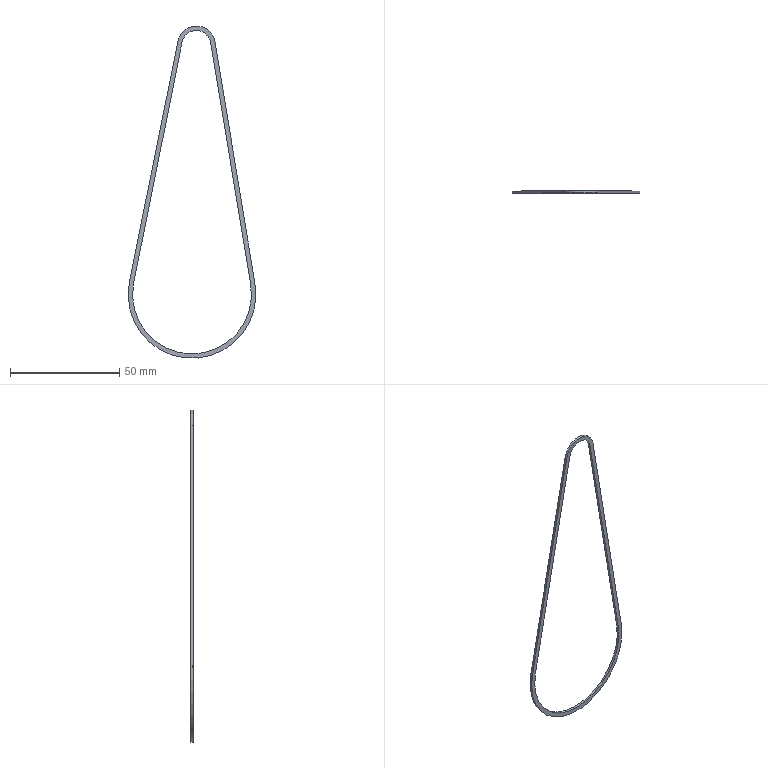Component | NX | MODEL9 | 1 solid | 13 faces | box 58.43 x 1 x 152.1 mm | volume 690 mm3 | plane 9 | cylinder 4 | commonest cylinder face diameters 13.245 x1 58.434 x1 17.245 x1 54.434 x1
STEP:
#1=CARTESIAN_POINT('',(0.,0.,0.));
#2=DIRECTION('',(0.,0.,1.));
#3=DIRECTION('',(1.,0.,0.));
#4=AXIS2_PLACEMENT_3D('',#1,#2,#3);
#5=CARTESIAN_POINT('',(-28.676,9.953,-108.889));
#6=VERTEX_POINT('',#5);
#7=CARTESIAN_POINT('',(-28.77,9.953,-109.381));
#8=VERTEX_POINT('',#7);
#9=CARTESIAN_POINT('',(-28.676,9.953,-108.889));
#10=DIRECTION('',(-0.1883,0.,-0.9821));
#11=VECTOR('',#10,1.);
#12=LINE('',#9,#11);
#13=CARTESIAN_POINT('',(-28.676,8.953,-108.889));
#14=DIRECTION('',(0.9821,0.,-0.1883));
#15=DIRECTION('',(0.1883,0.,0.9821));
#16=AXIS2_PLACEMENT_3D('',#13,#14,#15);
#17=PLANE('',#16);
#18=CARTESIAN_POINT('',(0.,-1.));
#19=DIRECTION('',(-1.,0.));
#20=VECTOR('',#19,1.);
#21=LINE('',#18,#20);
#22=(GEOMETRIC_REPRESENTATION_CONTEXT(2)PARAMETRIC_REPRESENTATION_CONTEXT()REPRESENTATION_CONTEXT('',''));
#23=DEFINITIONAL_REPRESENTATION('',(#21),#22);
#24=PCURVE('',#17,#23);
#25=CARTESIAN_POINT('',(-1.994,9.953,-114.26));
#26=DIRECTION('',(0.,-1.,0.));
#27=DIRECTION('',(1.,0.,0.));
#28=AXIS2_PLACEMENT_3D('',#25,#26,#27);
#29=PLANE('',#28);
#30=CARTESIAN_POINT('',(-26.682,5.371));
#31=DIRECTION('',(-0.1883,-0.9821));
#32=VECTOR('',#31,1.);
#33=LINE('',#30,#32);
#34=(GEOMETRIC_REPRESENTATION_CONTEXT(2)PARAMETRIC_REPRESENTATION_CONTEXT()REPRESENTATION_CONTEXT('',''));
#35=DEFINITIONAL_REPRESENTATION('',(#33),#34);
#36=PCURVE('',#29,#35);
#37=SURFACE_CURVE('',#12,(#24,#36),.PCURVE_S1.);
#38=EDGE_CURVE('',#6,#8,#37,.T.);
#39=ORIENTED_EDGE('',*,*,#38,.F.);
#40=CARTESIAN_POINT('',(-28.676,8.953,-108.889));
#41=VERTEX_POINT('',#40);
#42=CARTESIAN_POINT('',(-28.676,8.953,-108.889));
#43=DIRECTION('',(0.,1.,0.));
#44=VECTOR('',#43,1.);
#45=LINE('',#42,#44);
#46=CARTESIAN_POINT('',(0.,0.));
#47=DIRECTION('',(0.,-1.));
#48=VECTOR('',#47,1.);
#49=LINE('',#46,#48);
#50=(GEOMETRIC_REPRESENTATION_CONTEXT(2)PARAMETRIC_REPRESENTATION_CONTEXT()REPRESENTATION_CONTEXT('',''));
#51=DEFINITIONAL_REPRESENTATION('',(#49),#50);
#52=PCURVE('',#17,#51);
#53=CARTESIAN_POINT('',(-6.492,8.953,1.307));
#54=DIRECTION('',(0.9803,0.,-0.1974));
#55=DIRECTION('',(0.1974,0.,0.9803));
#56=AXIS2_PLACEMENT_3D('',#53,#54,#55);
#57=PLANE('',#56);
#58=CARTESIAN_POINT('',(-112.407,0.));
#59=DIRECTION('',(0.,-1.));
#60=VECTOR('',#59,1.);
#61=LINE('',#58,#60);
#62=(GEOMETRIC_REPRESENTATION_CONTEXT(2)PARAMETRIC_REPRESENTATION_CONTEXT()REPRESENTATION_CONTEXT('',''));
#63=DEFINITIONAL_REPRESENTATION('',(#61),#62);
#64=PCURVE('',#57,#63);
#65=SURFACE_CURVE('',#45,(#52,#64),.PCURVE_S1.);
#66=EDGE_CURVE('',#41,#6,#65,.T.);
#67=ORIENTED_EDGE('',*,*,#66,.F.);
#68=CARTESIAN_POINT('',(-28.77,8.953,-109.381));
#69=VERTEX_POINT('',#68);
#70=CARTESIAN_POINT('',(-28.676,8.953,-108.889));
#71=DIRECTION('',(-0.1883,0.,-0.9821));
#72=VECTOR('',#71,1.);
#73=LINE('',#70,#72);
#74=CARTESIAN_POINT('',(0.,0.));
#75=DIRECTION('',(-1.,0.));
#76=VECTOR('',#75,1.);
#77=LINE('',#74,#76);
#78=(GEOMETRIC_REPRESENTATION_CONTEXT(2)PARAMETRIC_REPRESENTATION_CONTEXT()REPRESENTATION_CONTEXT('',''));
#79=DEFINITIONAL_REPRESENTATION('',(#77),#78);
#80=PCURVE('',#17,#79);
#81=CARTESIAN_POINT('',(-1.994,8.953,-114.26));
#82=DIRECTION('',(0.,-1.,0.));
#83=DIRECTION('',(1.,0.,0.));
#84=AXIS2_PLACEMENT_3D('',#81,#82,#83);
#85=PLANE('',#84);
#86=CARTESIAN_POINT('',(-26.682,5.371));
#87=DIRECTION('',(-0.1883,-0.9821));
#88=VECTOR('',#87,1.);
#89=LINE('',#86,#88);
#90=(GEOMETRIC_REPRESENTATION_CONTEXT(2)PARAMETRIC_REPRESENTATION_CONTEXT()REPRESENTATION_CONTEXT('',''));
#91=DEFINITIONAL_REPRESENTATION('',(#89),#90);
#92=PCURVE('',#85,#91);
#93=SURFACE_CURVE('',#73,(#80,#92),.PCURVE_S1.);
#94=EDGE_CURVE('',#41,#69,#93,.T.);
#95=ORIENTED_EDGE('',*,*,#94,.T.);
#96=CARTESIAN_POINT('',(-28.77,8.953,-109.381));
#97=DIRECTION('',(0.,1.,0.));
#98=VECTOR('',#97,1.);
#99=LINE('',#96,#98);
#100=CARTESIAN_POINT('',(-0.5007,0.));
#101=DIRECTION('',(0.,-1.));
#102=VECTOR('',#101,1.);
#103=LINE('',#100,#102);
#104=(GEOMETRIC_REPRESENTATION_CONTEXT(2)PARAMETRIC_REPRESENTATION_CONTEXT()REPRESENTATION_CONTEXT('',''));
#105=DEFINITIONAL_REPRESENTATION('',(#103),#104);
#106=PCURVE('',#17,#105);
#107=CARTESIAN_POINT('',(-1.994,8.953,-114.26));
#108=DIRECTION('',(0.,1.,0.));
#109=DIRECTION('',(-1.,0.,0.));
#110=AXIS2_PLACEMENT_3D('',#107,#108,#109);
#111=CYLINDRICAL_SURFACE('',#110,27.217);
#112=CARTESIAN_POINT('',(6.463,0.));
#113=DIRECTION('',(0.,1.));
#114=VECTOR('',#113,1.);
#115=LINE('',#112,#114);
#116=(GEOMETRIC_REPRESENTATION_CONTEXT(2)PARAMETRIC_REPRESENTATION_CONTEXT()REPRESENTATION_CONTEXT('',''));
#117=DEFINITIONAL_REPRESENTATION('',(#115),#116);
#118=PCURVE('',#111,#117);
#119=SURFACE_CURVE('',#99,(#106,#118),.PCURVE_S1.);
#120=EDGE_CURVE('',#69,#8,#119,.T.);
#121=ORIENTED_EDGE('',*,*,#120,.T.);
#122=EDGE_LOOP('',(#39,#67,#95,#121));
#123=FACE_BOUND('',#122,.T.);
#124=ADVANCED_FACE('',(#123),#17,.T.);
#125=CARTESIAN_POINT('',(-6.492,9.953,1.307));
#126=VERTEX_POINT('',#125);
#127=CARTESIAN_POINT('',(-6.492,9.953,1.307));
#128=DIRECTION('',(-0.1974,0.,-0.9803));
#129=VECTOR('',#128,1.);
#130=LINE('',#127,#129);
#131=CARTESIAN_POINT('',(0.,-1.));
#132=DIRECTION('',(-1.,0.));
#133=VECTOR('',#132,1.);
#134=LINE('',#131,#133);
#135=(GEOMETRIC_REPRESENTATION_CONTEXT(2)PARAMETRIC_REPRESENTATION_CONTEXT()REPRESENTATION_CONTEXT('',''));
#136=DEFINITIONAL_REPRESENTATION('',(#134),#135);
#137=PCURVE('',#57,#136);
#138=CARTESIAN_POINT('',(-4.498,115.567));
#139=DIRECTION('',(-0.1974,-0.9803));
#140=VECTOR('',#139,1.);
#141=LINE('',#138,#140);
#142=(GEOMETRIC_REPRESENTATION_CONTEXT(2)PARAMETRIC_REPRESENTATION_CONTEXT()REPRESENTATION_CONTEXT('',''));
#143=DEFINITIONAL_REPRESENTATION('',(#141),#142);
#144=PCURVE('',#29,#143);
#145=SURFACE_CURVE('',#130,(#137,#144),.PCURVE_S1.);
#146=EDGE_CURVE('',#126,#6,#145,.T.);
#147=ORIENTED_EDGE('',*,*,#146,.F.);
#148=CARTESIAN_POINT('',(-6.492,8.953,1.307));
#149=VERTEX_POINT('',#148);
#150=CARTESIAN_POINT('',(-6.492,8.953,1.307));
#151=DIRECTION('',(0.,1.,0.));
#152=VECTOR('',#151,1.);
#153=LINE('',#150,#152);
#154=CARTESIAN_POINT('',(-0.,0.));
#155=DIRECTION('',(0.,-1.));
#156=VECTOR('',#155,1.);
#157=LINE('',#154,#156);
#158=(GEOMETRIC_REPRESENTATION_CONTEXT(2)PARAMETRIC_REPRESENTATION_CONTEXT()REPRESENTATION_CONTEXT('',''));
#159=DEFINITIONAL_REPRESENTATION('',(#157),#158);
#160=PCURVE('',#57,#159);
#161=CARTESIAN_POINT('',(0.,8.953,0.));
#162=DIRECTION('',(0.,1.,0.));
#163=DIRECTION('',(-1.,0.,0.));
#164=AXIS2_PLACEMENT_3D('',#161,#162,#163);
#165=CYLINDRICAL_SURFACE('',#164,6.622);
#166=CARTESIAN_POINT('',(0.1987,0.));
#167=DIRECTION('',(0.,1.));
#168=VECTOR('',#167,1.);
#169=LINE('',#166,#168);
#170=(GEOMETRIC_REPRESENTATION_CONTEXT(2)PARAMETRIC_REPRESENTATION_CONTEXT()REPRESENTATION_CONTEXT('',''));
#171=DEFINITIONAL_REPRESENTATION('',(#169),#170);
#172=PCURVE('',#165,#171);
#173=SURFACE_CURVE('',#153,(#160,#172),.PCURVE_S1.);
#174=EDGE_CURVE('',#149,#126,#173,.T.);
#175=ORIENTED_EDGE('',*,*,#174,.F.);
#176=CARTESIAN_POINT('',(-6.492,8.953,1.307));
#177=DIRECTION('',(-0.1974,0.,-0.9803));
#178=VECTOR('',#177,1.);
#179=LINE('',#176,#178);
#180=CARTESIAN_POINT('',(0.,0.));
#181=DIRECTION('',(-1.,0.));
#182=VECTOR('',#181,1.);
#183=LINE('',#180,#182);
#184=(GEOMETRIC_REPRESENTATION_CONTEXT(2)PARAMETRIC_REPRESENTATION_CONTEXT()REPRESENTATION_CONTEXT('',''));
#185=DEFINITIONAL_REPRESENTATION('',(#183),#184);
#186=PCURVE('',#57,#185);
#187=CARTESIAN_POINT('',(-4.498,115.567));
#188=DIRECTION('',(-0.1974,-0.9803));
#189=VECTOR('',#188,1.);
#190=LINE('',#187,#189);
#191=(GEOMETRIC_REPRESENTATION_CONTEXT(2)PARAMETRIC_REPRESENTATION_CONTEXT()REPRESENTATION_CONTEXT('',''));
#192=DEFINITIONAL_REPRESENTATION('',(#190),#191);
#193=PCURVE('',#85,#192);
#194=SURFACE_CURVE('',#179,(#186,#193),.PCURVE_S1.);
#195=EDGE_CURVE('',#149,#41,#194,.T.);
#196=ORIENTED_EDGE('',*,*,#195,.T.);
#197=ORIENTED_EDGE('',*,*,#66,.T.);
#198=EDGE_LOOP('',(#147,#175,#196,#197));
#199=FACE_BOUND('',#198,.T.);
#200=ADVANCED_FACE('',(#199),#57,.T.);
#201=ORIENTED_EDGE('',*,*,#174,.F.);
#202=CARTESIAN_POINT('',(6.534,8.953,1.08));
#203=VERTEX_POINT('',#202);
#204=CARTESIAN_POINT('',(0.,8.953,0.));
#205=DIRECTION('',(0.,-1.,0.));
#206=DIRECTION('',(1.,0.,0.));
#207=AXIS2_PLACEMENT_3D('',#204,#205,#206);
#208=CIRCLE('',#207,6.622);
#209=CARTESIAN_POINT('',(3.142,0.));
#210=DIRECTION('',(-1.,0.));
#211=VECTOR('',#210,1.);
#212=LINE('',#209,#211);
#213=(GEOMETRIC_REPRESENTATION_CONTEXT(2)PARAMETRIC_REPRESENTATION_CONTEXT()REPRESENTATION_CONTEXT('',''));
#214=DEFINITIONAL_REPRESENTATION('',(#212),#213);
#215=PCURVE('',#165,#214);
#216=CARTESIAN_POINT('',(1.994,114.26));
#217=DIRECTION('',(1.,0.));
#218=AXIS2_PLACEMENT_2D('',#216,#217);
#219=CIRCLE('',#218,6.622);
#220=(GEOMETRIC_REPRESENTATION_CONTEXT(2)PARAMETRIC_REPRESENTATION_CONTEXT()REPRESENTATION_CONTEXT('',''));
#221=DEFINITIONAL_REPRESENTATION('',(#219),#220);
#222=PCURVE('',#85,#221);
#223=SURFACE_CURVE('',#208,(#215,#222),.PCURVE_S1.);
#224=EDGE_CURVE('',#203,#149,#223,.T.);
#225=ORIENTED_EDGE('',*,*,#224,.F.);
#226=CARTESIAN_POINT('',(6.534,9.953,1.08));
#227=VERTEX_POINT('',#226);
#228=CARTESIAN_POINT('',(6.534,8.953,1.08));
#229=DIRECTION('',(0.,1.,0.));
#230=VECTOR('',#229,1.);
#231=LINE('',#228,#230);
#232=CARTESIAN_POINT('',(2.978,0.));
#233=DIRECTION('',(0.,1.));
#234=VECTOR('',#233,1.);
#235=LINE('',#232,#234);
#236=(GEOMETRIC_REPRESENTATION_CONTEXT(2)PARAMETRIC_REPRESENTATION_CONTEXT()REPRESENTATION_CONTEXT('',''));
#237=DEFINITIONAL_REPRESENTATION('',(#235),#236);
#238=PCURVE('',#165,#237);
#239=CARTESIAN_POINT('',(24.858,8.953,-109.823));
#240=DIRECTION('',(-0.9866,0.,-0.163));
#241=DIRECTION('',(0.163,0.,-0.9866));
#242=AXIS2_PLACEMENT_3D('',#239,#240,#241);
#243=PLANE('',#242);
#244=CARTESIAN_POINT('',(-112.407,0.));
#245=DIRECTION('',(0.,-1.));
#246=VECTOR('',#245,1.);
#247=LINE('',#244,#246);
#248=(GEOMETRIC_REPRESENTATION_CONTEXT(2)PARAMETRIC_REPRESENTATION_CONTEXT()REPRESENTATION_CONTEXT('',''));
#249=DEFINITIONAL_REPRESENTATION('',(#247),#248);
#250=PCURVE('',#243,#249);
#251=SURFACE_CURVE('',#231,(#238,#250),.PCURVE_S1.);
#252=EDGE_CURVE('',#203,#227,#251,.T.);
#253=ORIENTED_EDGE('',*,*,#252,.T.);
#254=CARTESIAN_POINT('',(0.,9.953,0.));
#255=DIRECTION('',(0.,-1.,0.));
#256=DIRECTION('',(1.,0.,0.));
#257=AXIS2_PLACEMENT_3D('',#254,#255,#256);
#258=CIRCLE('',#257,6.622);
#259=CARTESIAN_POINT('',(3.142,1.));
#260=DIRECTION('',(-1.,0.));
#261=VECTOR('',#260,1.);
#262=LINE('',#259,#261);
#263=(GEOMETRIC_REPRESENTATION_CONTEXT(2)PARAMETRIC_REPRESENTATION_CONTEXT()REPRESENTATION_CONTEXT('',''));
#264=DEFINITIONAL_REPRESENTATION('',(#262),#263);
#265=PCURVE('',#165,#264);
#266=CARTESIAN_POINT('',(1.994,114.26));
#267=DIRECTION('',(1.,0.));
#268=AXIS2_PLACEMENT_2D('',#266,#267);
#269=CIRCLE('',#268,6.622);
#270=(GEOMETRIC_REPRESENTATION_CONTEXT(2)PARAMETRIC_REPRESENTATION_CONTEXT()REPRESENTATION_CONTEXT('',''));
#271=DEFINITIONAL_REPRESENTATION('',(#269),#270);
#272=PCURVE('',#29,#271);
#273=SURFACE_CURVE('',#258,(#265,#272),.PCURVE_S1.);
#274=EDGE_CURVE('',#227,#126,#273,.T.);
#275=ORIENTED_EDGE('',*,*,#274,.T.);
#276=EDGE_LOOP('',(#201,#225,#253,#275));
#277=FACE_BOUND('',#276,.F.);
#278=ADVANCED_FACE('',(#277),#165,.F.);
#279=CARTESIAN_POINT('',(24.858,9.953,-109.823));
#280=VERTEX_POINT('',#279);
#281=CARTESIAN_POINT('',(24.858,9.953,-109.823));
#282=DIRECTION('',(-0.163,0.,0.9866));
#283=VECTOR('',#282,1.);
#284=LINE('',#281,#283);
#285=CARTESIAN_POINT('',(0.,-1.));
#286=DIRECTION('',(-1.,0.));
#287=VECTOR('',#286,1.);
#288=LINE('',#285,#287);
#289=(GEOMETRIC_REPRESENTATION_CONTEXT(2)PARAMETRIC_REPRESENTATION_CONTEXT()REPRESENTATION_CONTEXT('',''));
#290=DEFINITIONAL_REPRESENTATION('',(#288),#289);
#291=PCURVE('',#243,#290);
#292=CARTESIAN_POINT('',(26.853,4.437));
#293=DIRECTION('',(-0.163,0.9866));
#294=VECTOR('',#293,1.);
#295=LINE('',#292,#294);
#296=(GEOMETRIC_REPRESENTATION_CONTEXT(2)PARAMETRIC_REPRESENTATION_CONTEXT()REPRESENTATION_CONTEXT('',''));
#297=DEFINITIONAL_REPRESENTATION('',(#295),#296);
#298=PCURVE('',#29,#297);
#299=SURFACE_CURVE('',#284,(#291,#298),.PCURVE_S1.);
#300=EDGE_CURVE('',#280,#227,#299,.T.);
#301=ORIENTED_EDGE('',*,*,#300,.F.);
#302=CARTESIAN_POINT('',(24.858,8.953,-109.823));
#303=VERTEX_POINT('',#302);
#304=CARTESIAN_POINT('',(24.858,8.953,-109.823));
#305=DIRECTION('',(0.,1.,0.));
#306=VECTOR('',#305,1.);
#307=LINE('',#304,#306);
#308=CARTESIAN_POINT('',(0.,0.));
#309=DIRECTION('',(0.,-1.));
#310=VECTOR('',#309,1.);
#311=LINE('',#308,#310);
#312=(GEOMETRIC_REPRESENTATION_CONTEXT(2)PARAMETRIC_REPRESENTATION_CONTEXT()REPRESENTATION_CONTEXT('',''));
#313=DEFINITIONAL_REPRESENTATION('',(#311),#312);
#314=PCURVE('',#243,#313);
#315=CARTESIAN_POINT('',(2.978,0.));
#316=DIRECTION('',(0.,1.));
#317=VECTOR('',#316,1.);
#318=LINE('',#315,#317);
#319=(GEOMETRIC_REPRESENTATION_CONTEXT(2)PARAMETRIC_REPRESENTATION_CONTEXT()REPRESENTATION_CONTEXT('',''));
#320=DEFINITIONAL_REPRESENTATION('',(#318),#319);
#321=PCURVE('',#111,#320);
#322=SURFACE_CURVE('',#307,(#314,#321),.PCURVE_S1.);
#323=EDGE_CURVE('',#303,#280,#322,.T.);
#324=ORIENTED_EDGE('',*,*,#323,.F.);
#325=CARTESIAN_POINT('',(24.858,8.953,-109.823));
#326=DIRECTION('',(-0.163,0.,0.9866));
#327=VECTOR('',#326,1.);
#328=LINE('',#325,#327);
#329=CARTESIAN_POINT('',(0.,0.));
#330=DIRECTION('',(-1.,0.));
#331=VECTOR('',#330,1.);
#332=LINE('',#329,#331);
#333=(GEOMETRIC_REPRESENTATION_CONTEXT(2)PARAMETRIC_REPRESENTATION_CONTEXT()REPRESENTATION_CONTEXT('',''));
#334=DEFINITIONAL_REPRESENTATION('',(#332),#333);
#335=PCURVE('',#243,#334);
#336=CARTESIAN_POINT('',(26.853,4.437));
#337=DIRECTION('',(-0.163,0.9866));
#338=VECTOR('',#337,1.);
#339=LINE('',#336,#338);
#340=(GEOMETRIC_REPRESENTATION_CONTEXT(2)PARAMETRIC_REPRESENTATION_CONTEXT()REPRESENTATION_CONTEXT('',''));
#341=DEFINITIONAL_REPRESENTATION('',(#339),#340);
#342=PCURVE('',#85,#341);
#343=SURFACE_CURVE('',#328,(#335,#342),.PCURVE_S1.);
#344=EDGE_CURVE('',#303,#203,#343,.T.);
#345=ORIENTED_EDGE('',*,*,#344,.T.);
#346=ORIENTED_EDGE('',*,*,#252,.T.);
#347=EDGE_LOOP('',(#301,#324,#345,#346));
#348=FACE_BOUND('',#347,.T.);
#349=ADVANCED_FACE('',(#348),#243,.T.);
#350=CARTESIAN_POINT('',(-8.453,9.953,1.702));
#351=VERTEX_POINT('',#350);
#352=CARTESIAN_POINT('',(-30.639,9.953,-108.503));
#353=VERTEX_POINT('',#352);
#354=CARTESIAN_POINT('',(-8.453,9.953,1.702));
#355=DIRECTION('',(-0.1974,0.,-0.9803));
#356=VECTOR('',#355,1.);
#357=LINE('',#354,#356);
#358=CARTESIAN_POINT('',(-8.453,8.953,1.702));
#359=DIRECTION('',(0.9803,0.,-0.1974));
#360=DIRECTION('',(0.1974,0.,0.9803));
#361=AXIS2_PLACEMENT_3D('',#358,#359,#360);
#362=PLANE('',#361);
#363=CARTESIAN_POINT('',(0.,-1.));
#364=DIRECTION('',(-1.,0.));
#365=VECTOR('',#364,1.);
#366=LINE('',#363,#365);
#367=(GEOMETRIC_REPRESENTATION_CONTEXT(2)PARAMETRIC_REPRESENTATION_CONTEXT()REPRESENTATION_CONTEXT('',''));
#368=DEFINITIONAL_REPRESENTATION('',(#366),#367);
#369=PCURVE('',#362,#368);
#370=CARTESIAN_POINT('',(-6.458,115.962));
#371=DIRECTION('',(-0.1974,-0.9803));
#372=VECTOR('',#371,1.);
#373=LINE('',#370,#372);
#374=(GEOMETRIC_REPRESENTATION_CONTEXT(2)PARAMETRIC_REPRESENTATION_CONTEXT()REPRESENTATION_CONTEXT('',''));
#375=DEFINITIONAL_REPRESENTATION('',(#373),#374);
#376=PCURVE('',#29,#375);
#377=SURFACE_CURVE('',#357,(#369,#376),.PCURVE_S1.);
#378=EDGE_CURVE('',#351,#353,#377,.T.);
#379=ORIENTED_EDGE('',*,*,#378,.T.);
#380=CARTESIAN_POINT('',(-30.639,8.953,-108.503));
#381=VERTEX_POINT('',#380);
#382=CARTESIAN_POINT('',(-30.639,8.953,-108.503));
#383=DIRECTION('',(0.,1.,0.));
#384=VECTOR('',#383,1.);
#385=LINE('',#382,#384);
#386=CARTESIAN_POINT('',(-112.416,0.));
#387=DIRECTION('',(0.,-1.));
#388=VECTOR('',#387,1.);
#389=LINE('',#386,#388);
#390=(GEOMETRIC_REPRESENTATION_CONTEXT(2)PARAMETRIC_REPRESENTATION_CONTEXT()REPRESENTATION_CONTEXT('',''));
#391=DEFINITIONAL_REPRESENTATION('',(#389),#390);
#392=PCURVE('',#362,#391);
#393=CARTESIAN_POINT('',(-30.639,8.953,-108.503));
#394=DIRECTION('',(0.9821,0.,-0.1883));
#395=DIRECTION('',(0.1883,0.,0.9821));
#396=AXIS2_PLACEMENT_3D('',#393,#394,#395);
#397=PLANE('',#396);
#398=CARTESIAN_POINT('',(0.,0.));
#399=DIRECTION('',(0.,-1.));
#400=VECTOR('',#399,1.);
#401=LINE('',#398,#400);
#402=(GEOMETRIC_REPRESENTATION_CONTEXT(2)PARAMETRIC_REPRESENTATION_CONTEXT()REPRESENTATION_CONTEXT('',''));
#403=DEFINITIONAL_REPRESENTATION('',(#401),#402);
#404=PCURVE('',#397,#403);
#405=SURFACE_CURVE('',#385,(#392,#404),.PCURVE_S1.);
#406=EDGE_CURVE('',#381,#353,#405,.T.);
#407=ORIENTED_EDGE('',*,*,#406,.F.);
#408=CARTESIAN_POINT('',(-8.453,8.953,1.702));
#409=VERTEX_POINT('',#408);
#410=CARTESIAN_POINT('',(-8.453,8.953,1.702));
#411=DIRECTION('',(-0.1974,0.,-0.9803));
#412=VECTOR('',#411,1.);
#413=LINE('',#410,#412);
#414=CARTESIAN_POINT('',(0.,0.));
#415=DIRECTION('',(-1.,0.));
#416=VECTOR('',#415,1.);
#417=LINE('',#414,#416);
#418=(GEOMETRIC_REPRESENTATION_CONTEXT(2)PARAMETRIC_REPRESENTATION_CONTEXT()REPRESENTATION_CONTEXT('',''));
#419=DEFINITIONAL_REPRESENTATION('',(#417),#418);
#420=PCURVE('',#362,#419);
#421=CARTESIAN_POINT('',(-6.458,115.962));
#422=DIRECTION('',(-0.1974,-0.9803));
#423=VECTOR('',#422,1.);
#424=LINE('',#421,#423);
#425=(GEOMETRIC_REPRESENTATION_CONTEXT(2)PARAMETRIC_REPRESENTATION_CONTEXT()REPRESENTATION_CONTEXT('',''));
#426=DEFINITIONAL_REPRESENTATION('',(#424),#425);
#427=PCURVE('',#85,#426);
#428=SURFACE_CURVE('',#413,(#420,#427),.PCURVE_S1.);
#429=EDGE_CURVE('',#409,#381,#428,.T.);
#430=ORIENTED_EDGE('',*,*,#429,.F.);
#431=CARTESIAN_POINT('',(-8.453,8.953,1.702));
#432=DIRECTION('',(0.,1.,0.));
#433=VECTOR('',#432,1.);
#434=LINE('',#431,#433);
#435=CARTESIAN_POINT('',(0.,0.));
#436=DIRECTION('',(0.,-1.));
#437=VECTOR('',#436,1.);
#438=LINE('',#435,#437);
#439=(GEOMETRIC_REPRESENTATION_CONTEXT(2)PARAMETRIC_REPRESENTATION_CONTEXT()REPRESENTATION_CONTEXT('',''));
#440=DEFINITIONAL_REPRESENTATION('',(#438),#439);
#441=PCURVE('',#362,#440);
#442=CARTESIAN_POINT('',(0.,8.953,0.));
#443=DIRECTION('',(0.,1.,0.));
#444=DIRECTION('',(-1.,0.,0.));
#445=AXIS2_PLACEMENT_3D('',#442,#443,#444);
#446=CYLINDRICAL_SURFACE('',#445,8.623);
#447=CARTESIAN_POINT('',(0.1987,0.));
#448=DIRECTION('',(0.,1.));
#449=VECTOR('',#448,1.);
#450=LINE('',#447,#449);
#451=(GEOMETRIC_REPRESENTATION_CONTEXT(2)PARAMETRIC_REPRESENTATION_CONTEXT()REPRESENTATION_CONTEXT('',''));
#452=DEFINITIONAL_REPRESENTATION('',(#450),#451);
#453=PCURVE('',#446,#452);
#454=SURFACE_CURVE('',#434,(#441,#453),.PCURVE_S1.);
#455=EDGE_CURVE('',#409,#351,#454,.T.);
#456=ORIENTED_EDGE('',*,*,#455,.T.);
#457=EDGE_LOOP('',(#379,#407,#430,#456));
#458=FACE_BOUND('',#457,.T.);
#459=ADVANCED_FACE('',(#458),#362,.F.);
#460=CARTESIAN_POINT('',(-30.736,9.953,-109.013));
#461=VERTEX_POINT('',#460);
#462=CARTESIAN_POINT('',(-30.639,9.953,-108.503));
#463=DIRECTION('',(-0.1883,0.,-0.9821));
#464=VECTOR('',#463,1.);
#465=LINE('',#462,#464);
#466=CARTESIAN_POINT('',(0.,-1.));
#467=DIRECTION('',(-1.,0.));
#468=VECTOR('',#467,1.);
#469=LINE('',#466,#468);
#470=(GEOMETRIC_REPRESENTATION_CONTEXT(2)PARAMETRIC_REPRESENTATION_CONTEXT()REPRESENTATION_CONTEXT('',''));
#471=DEFINITIONAL_REPRESENTATION('',(#469),#470);
#472=PCURVE('',#397,#471);
#473=CARTESIAN_POINT('',(-28.644,5.757));
#474=DIRECTION('',(-0.1883,-0.9821));
#475=VECTOR('',#474,1.);
#476=LINE('',#473,#475);
#477=(GEOMETRIC_REPRESENTATION_CONTEXT(2)PARAMETRIC_REPRESENTATION_CONTEXT()REPRESENTATION_CONTEXT('',''));
#478=DEFINITIONAL_REPRESENTATION('',(#476),#477);
#479=PCURVE('',#29,#478);
#480=SURFACE_CURVE('',#465,(#472,#479),.PCURVE_S1.);
#481=EDGE_CURVE('',#353,#461,#480,.T.);
#482=ORIENTED_EDGE('',*,*,#481,.T.);
#483=CARTESIAN_POINT('',(-30.736,8.953,-109.013));
#484=VERTEX_POINT('',#483);
#485=CARTESIAN_POINT('',(-30.736,8.953,-109.013));
#486=DIRECTION('',(0.,1.,0.));
#487=VECTOR('',#486,1.);
#488=LINE('',#485,#487);
#489=CARTESIAN_POINT('',(-0.5191,0.));
#490=DIRECTION('',(0.,-1.));
#491=VECTOR('',#490,1.);
#492=LINE('',#489,#491);
#493=(GEOMETRIC_REPRESENTATION_CONTEXT(2)PARAMETRIC_REPRESENTATION_CONTEXT()REPRESENTATION_CONTEXT('',''));
#494=DEFINITIONAL_REPRESENTATION('',(#492),#493);
#495=PCURVE('',#397,#494);
#496=CARTESIAN_POINT('',(-30.736,8.953,-109.013));
#497=DIRECTION('',(0.9838,0.,-0.1793));
#498=DIRECTION('',(0.1793,0.,0.9838));
#499=AXIS2_PLACEMENT_3D('',#496,#497,#498);
#500=PLANE('',#499);
#501=CARTESIAN_POINT('',(0.,0.));
#502=DIRECTION('',(0.,-1.));
#503=VECTOR('',#502,1.);
#504=LINE('',#501,#503);
#505=(GEOMETRIC_REPRESENTATION_CONTEXT(2)PARAMETRIC_REPRESENTATION_CONTEXT()REPRESENTATION_CONTEXT('',''));
#506=DEFINITIONAL_REPRESENTATION('',(#504),#505);
#507=PCURVE('',#500,#506);
#508=SURFACE_CURVE('',#488,(#495,#507),.PCURVE_S1.);
#509=EDGE_CURVE('',#484,#461,#508,.T.);
#510=ORIENTED_EDGE('',*,*,#509,.F.);
#511=CARTESIAN_POINT('',(-30.639,8.953,-108.503));
#512=DIRECTION('',(-0.1883,0.,-0.9821));
#513=VECTOR('',#512,1.);
#514=LINE('',#511,#513);
#515=CARTESIAN_POINT('',(0.,0.));
#516=DIRECTION('',(-1.,0.));
#517=VECTOR('',#516,1.);
#518=LINE('',#515,#517);
#519=(GEOMETRIC_REPRESENTATION_CONTEXT(2)PARAMETRIC_REPRESENTATION_CONTEXT()REPRESENTATION_CONTEXT('',''));
#520=DEFINITIONAL_REPRESENTATION('',(#518),#519);
#521=PCURVE('',#397,#520);
#522=CARTESIAN_POINT('',(-28.644,5.757));
#523=DIRECTION('',(-0.1883,-0.9821));
#524=VECTOR('',#523,1.);
#525=LINE('',#522,#524);
#526=(GEOMETRIC_REPRESENTATION_CONTEXT(2)PARAMETRIC_REPRESENTATION_CONTEXT()REPRESENTATION_CONTEXT('',''));
#527=DEFINITIONAL_REPRESENTATION('',(#525),#526);
#528=PCURVE('',#85,#527);
#529=SURFACE_CURVE('',#514,(#521,#528),.PCURVE_S1.);
#530=EDGE_CURVE('',#381,#484,#529,.T.);
#531=ORIENTED_EDGE('',*,*,#530,.F.);
#532=ORIENTED_EDGE('',*,*,#406,.T.);
#533=EDGE_LOOP('',(#482,#510,#531,#532));
#534=FACE_BOUND('',#533,.T.);
#535=ADVANCED_FACE('',(#534),#397,.F.);
#536=CARTESIAN_POINT('',(-30.738,9.953,-109.022));
#537=VERTEX_POINT('',#536);
#538=CARTESIAN_POINT('',(-30.736,9.953,-109.013));
#539=DIRECTION('',(-0.1793,0.,-0.9838));
#540=VECTOR('',#539,1.);
#541=LINE('',#538,#540);
#542=CARTESIAN_POINT('',(0.,-1.));
#543=DIRECTION('',(-1.,0.));
#544=VECTOR('',#543,1.);
#545=LINE('',#542,#544);
#546=(GEOMETRIC_REPRESENTATION_CONTEXT(2)PARAMETRIC_REPRESENTATION_CONTEXT()REPRESENTATION_CONTEXT('',''));
#547=DEFINITIONAL_REPRESENTATION('',(#545),#546);
#548=PCURVE('',#500,#547);
#549=CARTESIAN_POINT('',(-28.742,5.247));
#550=DIRECTION('',(-0.1793,-0.9838));
#551=VECTOR('',#550,1.);
#552=LINE('',#549,#551);
#553=(GEOMETRIC_REPRESENTATION_CONTEXT(2)PARAMETRIC_REPRESENTATION_CONTEXT()REPRESENTATION_CONTEXT('',''));
#554=DEFINITIONAL_REPRESENTATION('',(#552),#553);
#555=PCURVE('',#29,#554);
#556=SURFACE_CURVE('',#541,(#548,#555),.PCURVE_S1.);
#557=EDGE_CURVE('',#461,#537,#556,.T.);
#558=ORIENTED_EDGE('',*,*,#557,.T.);
#559=CARTESIAN_POINT('',(-30.738,8.953,-109.022));
#560=VERTEX_POINT('',#559);
#561=CARTESIAN_POINT('',(-30.738,8.953,-109.022));
#562=DIRECTION('',(0.,1.,0.));
#563=VECTOR('',#562,1.);
#564=LINE('',#561,#563);
#565=CARTESIAN_POINT('',(-0.009199,0.));
#566=DIRECTION('',(0.,-1.));
#567=VECTOR('',#566,1.);
#568=LINE('',#565,#567);
#569=(GEOMETRIC_REPRESENTATION_CONTEXT(2)PARAMETRIC_REPRESENTATION_CONTEXT()REPRESENTATION_CONTEXT('',''));
#570=DEFINITIONAL_REPRESENTATION('',(#568),#569);
#571=PCURVE('',#500,#570);
#572=CARTESIAN_POINT('',(-1.994,8.953,-114.26));
#573=DIRECTION('',(0.,1.,0.));
#574=DIRECTION('',(-1.,0.,0.));
#575=AXIS2_PLACEMENT_3D('',#572,#573,#574);
#576=CYLINDRICAL_SURFACE('',#575,29.217);
#577=CARTESIAN_POINT('',(6.463,0.));
#578=DIRECTION('',(0.,1.));
#579=VECTOR('',#578,1.);
#580=LINE('',#577,#579);
#581=(GEOMETRIC_REPRESENTATION_CONTEXT(2)PARAMETRIC_REPRESENTATION_CONTEXT()REPRESENTATION_CONTEXT('',''));
#582=DEFINITIONAL_REPRESENTATION('',(#580),#581);
#583=PCURVE('',#576,#582);
#584=SURFACE_CURVE('',#564,(#571,#583),.PCURVE_S1.);
#585=EDGE_CURVE('',#560,#537,#584,.T.);
#586=ORIENTED_EDGE('',*,*,#585,.F.);
#587=CARTESIAN_POINT('',(-30.736,8.953,-109.013));
#588=DIRECTION('',(-0.1793,0.,-0.9838));
#589=VECTOR('',#588,1.);
#590=LINE('',#587,#589);
#591=CARTESIAN_POINT('',(0.,0.));
#592=DIRECTION('',(-1.,0.));
#593=VECTOR('',#592,1.);
#594=LINE('',#591,#593);
#595=(GEOMETRIC_REPRESENTATION_CONTEXT(2)PARAMETRIC_REPRESENTATION_CONTEXT()REPRESENTATION_CONTEXT('',''));
#596=DEFINITIONAL_REPRESENTATION('',(#594),#595);
#597=PCURVE('',#500,#596);
#598=CARTESIAN_POINT('',(-28.742,5.247));
#599=DIRECTION('',(-0.1793,-0.9838));
#600=VECTOR('',#599,1.);
#601=LINE('',#598,#600);
#602=(GEOMETRIC_REPRESENTATION_CONTEXT(2)PARAMETRIC_REPRESENTATION_CONTEXT()REPRESENTATION_CONTEXT('',''));
#603=DEFINITIONAL_REPRESENTATION('',(#601),#602);
#604=PCURVE('',#85,#603);
#605=SURFACE_CURVE('',#590,(#597,#604),.PCURVE_S1.);
#606=EDGE_CURVE('',#484,#560,#605,.T.);
#607=ORIENTED_EDGE('',*,*,#606,.F.);
#608=ORIENTED_EDGE('',*,*,#509,.T.);
#609=EDGE_LOOP('',(#558,#586,#607,#608));
#610=FACE_BOUND('',#609,.T.);
#611=ADVANCED_FACE('',(#610),#500,.F.);
#612=CARTESIAN_POINT('',(26.832,9.953,-109.497));
#613=VERTEX_POINT('',#612);
#614=CARTESIAN_POINT('',(-1.994,9.953,-114.26));
#615=DIRECTION('',(0.,-1.,0.));
#616=DIRECTION('',(1.,0.,0.));
#617=AXIS2_PLACEMENT_3D('',#614,#615,#616);
#618=CIRCLE('',#617,29.217);
#619=CARTESIAN_POINT('',(9.425,1.));
#620=DIRECTION('',(-1.,0.));
#621=VECTOR('',#620,1.);
#622=LINE('',#619,#621);
#623=(GEOMETRIC_REPRESENTATION_CONTEXT(2)PARAMETRIC_REPRESENTATION_CONTEXT()REPRESENTATION_CONTEXT('',''));
#624=DEFINITIONAL_REPRESENTATION('',(#622),#623);
#625=PCURVE('',#576,#624);
#626=CARTESIAN_POINT('',(0.,0.));
#627=DIRECTION('',(1.,0.));
#628=AXIS2_PLACEMENT_2D('',#626,#627);
#629=CIRCLE('',#628,29.217);
#630=(GEOMETRIC_REPRESENTATION_CONTEXT(2)PARAMETRIC_REPRESENTATION_CONTEXT()REPRESENTATION_CONTEXT('',''));
#631=DEFINITIONAL_REPRESENTATION('',(#629),#630);
#632=PCURVE('',#29,#631);
#633=SURFACE_CURVE('',#618,(#625,#632),.PCURVE_S1.);
#634=EDGE_CURVE('',#537,#613,#633,.T.);
#635=ORIENTED_EDGE('',*,*,#634,.T.);
#636=CARTESIAN_POINT('',(26.832,8.953,-109.497));
#637=VERTEX_POINT('',#636);
#638=CARTESIAN_POINT('',(26.832,8.953,-109.497));
#639=DIRECTION('',(0.,1.,0.));
#640=VECTOR('',#639,1.);
#641=LINE('',#638,#640);
#642=CARTESIAN_POINT('',(2.978,0.));
#643=DIRECTION('',(0.,1.));
#644=VECTOR('',#643,1.);
#645=LINE('',#642,#644);
#646=(GEOMETRIC_REPRESENTATION_CONTEXT(2)PARAMETRIC_REPRESENTATION_CONTEXT()REPRESENTATION_CONTEXT('',''));
#647=DEFINITIONAL_REPRESENTATION('',(#645),#646);
#648=PCURVE('',#576,#647);
#649=CARTESIAN_POINT('',(26.832,8.953,-109.497));
#650=DIRECTION('',(-0.9866,0.,-0.163));
#651=DIRECTION('',(0.163,0.,-0.9866));
#652=AXIS2_PLACEMENT_3D('',#649,#650,#651);
#653=PLANE('',#652);
#654=CARTESIAN_POINT('',(0.,0.));
#655=DIRECTION('',(0.,-1.));
#656=VECTOR('',#655,1.);
#657=LINE('',#654,#656);
#658=(GEOMETRIC_REPRESENTATION_CONTEXT(2)PARAMETRIC_REPRESENTATION_CONTEXT()REPRESENTATION_CONTEXT('',''));
#659=DEFINITIONAL_REPRESENTATION('',(#657),#658);
#660=PCURVE('',#653,#659);
#661=SURFACE_CURVE('',#641,(#648,#660),.PCURVE_S1.);
#662=EDGE_CURVE('',#637,#613,#661,.T.);
#663=ORIENTED_EDGE('',*,*,#662,.F.);
#664=CARTESIAN_POINT('',(-1.994,8.953,-114.26));
#665=DIRECTION('',(0.,-1.,0.));
#666=DIRECTION('',(1.,0.,0.));
#667=AXIS2_PLACEMENT_3D('',#664,#665,#666);
#668=CIRCLE('',#667,29.217);
#669=CARTESIAN_POINT('',(9.425,0.));
#670=DIRECTION('',(-1.,0.));
#671=VECTOR('',#670,1.);
#672=LINE('',#669,#671);
#673=(GEOMETRIC_REPRESENTATION_CONTEXT(2)PARAMETRIC_REPRESENTATION_CONTEXT()REPRESENTATION_CONTEXT('',''));
#674=DEFINITIONAL_REPRESENTATION('',(#672),#673);
#675=PCURVE('',#576,#674);
#676=CARTESIAN_POINT('',(0.,0.));
#677=DIRECTION('',(1.,0.));
#678=AXIS2_PLACEMENT_2D('',#676,#677);
#679=CIRCLE('',#678,29.217);
#680=(GEOMETRIC_REPRESENTATION_CONTEXT(2)PARAMETRIC_REPRESENTATION_CONTEXT()REPRESENTATION_CONTEXT('',''));
#681=DEFINITIONAL_REPRESENTATION('',(#679),#680);
#682=PCURVE('',#85,#681);
#683=SURFACE_CURVE('',#668,(#675,#682),.PCURVE_S1.);
#684=EDGE_CURVE('',#560,#637,#683,.T.);
#685=ORIENTED_EDGE('',*,*,#684,.F.);
#686=ORIENTED_EDGE('',*,*,#585,.T.);
#687=EDGE_LOOP('',(#635,#663,#685,#686));
#688=FACE_BOUND('',#687,.T.);
#689=ADVANCED_FACE('',(#688),#576,.T.);
#690=CARTESIAN_POINT('',(8.507,9.953,1.406));
#691=VERTEX_POINT('',#690);
#692=CARTESIAN_POINT('',(26.832,9.953,-109.497));
#693=DIRECTION('',(-0.163,0.,0.9866));
#694=VECTOR('',#693,1.);
#695=LINE('',#692,#694);
#696=CARTESIAN_POINT('',(0.,-1.));
#697=DIRECTION('',(-1.,0.));
#698=VECTOR('',#697,1.);
#699=LINE('',#696,#698);
#700=(GEOMETRIC_REPRESENTATION_CONTEXT(2)PARAMETRIC_REPRESENTATION_CONTEXT()REPRESENTATION_CONTEXT('',''));
#701=DEFINITIONAL_REPRESENTATION('',(#699),#700);
#702=PCURVE('',#653,#701);
#703=CARTESIAN_POINT('',(28.826,4.763));
#704=DIRECTION('',(-0.163,0.9866));
#705=VECTOR('',#704,1.);
#706=LINE('',#703,#705);
#707=(GEOMETRIC_REPRESENTATION_CONTEXT(2)PARAMETRIC_REPRESENTATION_CONTEXT()REPRESENTATION_CONTEXT('',''));
#708=DEFINITIONAL_REPRESENTATION('',(#706),#707);
#709=PCURVE('',#29,#708);
#710=SURFACE_CURVE('',#695,(#702,#709),.PCURVE_S1.);
#711=EDGE_CURVE('',#613,#691,#710,.T.);
#712=ORIENTED_EDGE('',*,*,#711,.T.);
#713=CARTESIAN_POINT('',(8.507,8.953,1.406));
#714=VERTEX_POINT('',#713);
#715=CARTESIAN_POINT('',(8.507,8.953,1.406));
#716=DIRECTION('',(0.,1.,0.));
#717=VECTOR('',#716,1.);
#718=LINE('',#715,#717);
#719=CARTESIAN_POINT('',(-112.407,0.));
#720=DIRECTION('',(0.,-1.));
#721=VECTOR('',#720,1.);
#722=LINE('',#719,#721);
#723=(GEOMETRIC_REPRESENTATION_CONTEXT(2)PARAMETRIC_REPRESENTATION_CONTEXT()REPRESENTATION_CONTEXT('',''));
#724=DEFINITIONAL_REPRESENTATION('',(#722),#723);
#725=PCURVE('',#653,#724);
#726=CARTESIAN_POINT('',(2.978,0.));
#727=DIRECTION('',(0.,1.));
#728=VECTOR('',#727,1.);
#729=LINE('',#726,#728);
#730=(GEOMETRIC_REPRESENTATION_CONTEXT(2)PARAMETRIC_REPRESENTATION_CONTEXT()REPRESENTATION_CONTEXT('',''));
#731=DEFINITIONAL_REPRESENTATION('',(#729),#730);
#732=PCURVE('',#446,#731);
#733=SURFACE_CURVE('',#718,(#725,#732),.PCURVE_S1.);
#734=EDGE_CURVE('',#714,#691,#733,.T.);
#735=ORIENTED_EDGE('',*,*,#734,.F.);
#736=CARTESIAN_POINT('',(26.832,8.953,-109.497));
#737=DIRECTION('',(-0.163,0.,0.9866));
#738=VECTOR('',#737,1.);
#739=LINE('',#736,#738);
#740=CARTESIAN_POINT('',(0.,0.));
#741=DIRECTION('',(-1.,0.));
#742=VECTOR('',#741,1.);
#743=LINE('',#740,#742);
#744=(GEOMETRIC_REPRESENTATION_CONTEXT(2)PARAMETRIC_REPRESENTATION_CONTEXT()REPRESENTATION_CONTEXT('',''));
#745=DEFINITIONAL_REPRESENTATION('',(#743),#744);
#746=PCURVE('',#653,#745);
#747=CARTESIAN_POINT('',(28.826,4.763));
#748=DIRECTION('',(-0.163,0.9866));
#749=VECTOR('',#748,1.);
#750=LINE('',#747,#749);
#751=(GEOMETRIC_REPRESENTATION_CONTEXT(2)PARAMETRIC_REPRESENTATION_CONTEXT()REPRESENTATION_CONTEXT('',''));
#752=DEFINITIONAL_REPRESENTATION('',(#750),#751);
#753=PCURVE('',#85,#752);
#754=SURFACE_CURVE('',#739,(#746,#753),.PCURVE_S1.);
#755=EDGE_CURVE('',#637,#714,#754,.T.);
#756=ORIENTED_EDGE('',*,*,#755,.F.);
#757=ORIENTED_EDGE('',*,*,#662,.T.);
#758=EDGE_LOOP('',(#712,#735,#756,#757));
#759=FACE_BOUND('',#758,.T.);
#760=ADVANCED_FACE('',(#759),#653,.F.);
#761=CARTESIAN_POINT('',(0.,9.953,0.));
#762=DIRECTION('',(0.,-1.,0.));
#763=DIRECTION('',(1.,0.,0.));
#764=AXIS2_PLACEMENT_3D('',#761,#762,#763);
#765=CIRCLE('',#764,8.623);
#766=CARTESIAN_POINT('',(3.142,1.));
#767=DIRECTION('',(-1.,0.));
#768=VECTOR('',#767,1.);
#769=LINE('',#766,#768);
#770=(GEOMETRIC_REPRESENTATION_CONTEXT(2)PARAMETRIC_REPRESENTATION_CONTEXT()REPRESENTATION_CONTEXT('',''));
#771=DEFINITIONAL_REPRESENTATION('',(#769),#770);
#772=PCURVE('',#446,#771);
#773=CARTESIAN_POINT('',(1.994,114.26));
#774=DIRECTION('',(1.,0.));
#775=AXIS2_PLACEMENT_2D('',#773,#774);
#776=CIRCLE('',#775,8.623);
#777=(GEOMETRIC_REPRESENTATION_CONTEXT(2)PARAMETRIC_REPRESENTATION_CONTEXT()REPRESENTATION_CONTEXT('',''));
#778=DEFINITIONAL_REPRESENTATION('',(#776),#777);
#779=PCURVE('',#29,#778);
#780=SURFACE_CURVE('',#765,(#772,#779),.PCURVE_S1.);
#781=EDGE_CURVE('',#691,#351,#780,.T.);
#782=ORIENTED_EDGE('',*,*,#781,.T.);
#783=ORIENTED_EDGE('',*,*,#455,.F.);
#784=CARTESIAN_POINT('',(0.,8.953,0.));
#785=DIRECTION('',(0.,-1.,0.));
#786=DIRECTION('',(1.,0.,0.));
#787=AXIS2_PLACEMENT_3D('',#784,#785,#786);
#788=CIRCLE('',#787,8.623);
#789=CARTESIAN_POINT('',(3.142,0.));
#790=DIRECTION('',(-1.,0.));
#791=VECTOR('',#790,1.);
#792=LINE('',#789,#791);
#793=(GEOMETRIC_REPRESENTATION_CONTEXT(2)PARAMETRIC_REPRESENTATION_CONTEXT()REPRESENTATION_CONTEXT('',''));
#794=DEFINITIONAL_REPRESENTATION('',(#792),#793);
#795=PCURVE('',#446,#794);
#796=CARTESIAN_POINT('',(1.994,114.26));
#797=DIRECTION('',(1.,0.));
#798=AXIS2_PLACEMENT_2D('',#796,#797);
#799=CIRCLE('',#798,8.623);
#800=(GEOMETRIC_REPRESENTATION_CONTEXT(2)PARAMETRIC_REPRESENTATION_CONTEXT()REPRESENTATION_CONTEXT('',''));
#801=DEFINITIONAL_REPRESENTATION('',(#799),#800);
#802=PCURVE('',#85,#801);
#803=SURFACE_CURVE('',#788,(#795,#802),.PCURVE_S1.);
#804=EDGE_CURVE('',#714,#409,#803,.T.);
#805=ORIENTED_EDGE('',*,*,#804,.F.);
#806=ORIENTED_EDGE('',*,*,#734,.T.);
#807=EDGE_LOOP('',(#782,#783,#805,#806));
#808=FACE_BOUND('',#807,.T.);
#809=ADVANCED_FACE('',(#808),#446,.T.);
#810=ORIENTED_EDGE('',*,*,#323,.F.);
#811=CARTESIAN_POINT('',(-1.994,8.953,-114.26));
#812=DIRECTION('',(0.,-1.,0.));
#813=DIRECTION('',(1.,0.,0.));
#814=AXIS2_PLACEMENT_3D('',#811,#812,#813);
#815=CIRCLE('',#814,27.217);
#816=CARTESIAN_POINT('',(9.425,0.));
#817=DIRECTION('',(-1.,0.));
#818=VECTOR('',#817,1.);
#819=LINE('',#816,#818);
#820=(GEOMETRIC_REPRESENTATION_CONTEXT(2)PARAMETRIC_REPRESENTATION_CONTEXT()REPRESENTATION_CONTEXT('',''));
#821=DEFINITIONAL_REPRESENTATION('',(#819),#820);
#822=PCURVE('',#111,#821);
#823=CARTESIAN_POINT('',(0.,0.));
#824=DIRECTION('',(1.,0.));
#825=AXIS2_PLACEMENT_2D('',#823,#824);
#826=CIRCLE('',#825,27.217);
#827=(GEOMETRIC_REPRESENTATION_CONTEXT(2)PARAMETRIC_REPRESENTATION_CONTEXT()REPRESENTATION_CONTEXT('',''));
#828=DEFINITIONAL_REPRESENTATION('',(#826),#827);
#829=PCURVE('',#85,#828);
#830=SURFACE_CURVE('',#815,(#822,#829),.PCURVE_S1.);
#831=EDGE_CURVE('',#69,#303,#830,.T.);
#832=ORIENTED_EDGE('',*,*,#831,.F.);
#833=ORIENTED_EDGE('',*,*,#120,.T.);
#834=CARTESIAN_POINT('',(-1.994,9.953,-114.26));
#835=DIRECTION('',(0.,-1.,0.));
#836=DIRECTION('',(1.,0.,0.));
#837=AXIS2_PLACEMENT_3D('',#834,#835,#836);
#838=CIRCLE('',#837,27.217);
#839=CARTESIAN_POINT('',(9.425,1.));
#840=DIRECTION('',(-1.,0.));
#841=VECTOR('',#840,1.);
#842=LINE('',#839,#841);
#843=(GEOMETRIC_REPRESENTATION_CONTEXT(2)PARAMETRIC_REPRESENTATION_CONTEXT()REPRESENTATION_CONTEXT('',''));
#844=DEFINITIONAL_REPRESENTATION('',(#842),#843);
#845=PCURVE('',#111,#844);
#846=CARTESIAN_POINT('',(0.,0.));
#847=DIRECTION('',(1.,0.));
#848=AXIS2_PLACEMENT_2D('',#846,#847);
#849=CIRCLE('',#848,27.217);
#850=(GEOMETRIC_REPRESENTATION_CONTEXT(2)PARAMETRIC_REPRESENTATION_CONTEXT()REPRESENTATION_CONTEXT('',''));
#851=DEFINITIONAL_REPRESENTATION('',(#849),#850);
#852=PCURVE('',#29,#851);
#853=SURFACE_CURVE('',#838,(#845,#852),.PCURVE_S1.);
#854=EDGE_CURVE('',#8,#280,#853,.T.);
#855=ORIENTED_EDGE('',*,*,#854,.T.);
#856=EDGE_LOOP('',(#810,#832,#833,#855));
#857=FACE_BOUND('',#856,.F.);
#858=ADVANCED_FACE('',(#857),#111,.F.);
#859=ORIENTED_EDGE('',*,*,#429,.T.);
#860=ORIENTED_EDGE('',*,*,#530,.T.);
#861=ORIENTED_EDGE('',*,*,#606,.T.);
#862=ORIENTED_EDGE('',*,*,#684,.T.);
#863=ORIENTED_EDGE('',*,*,#755,.T.);
#864=ORIENTED_EDGE('',*,*,#804,.T.);
#865=EDGE_LOOP('',(#859,#860,#861,#862,#863,#864));
#866=FACE_BOUND('',#865,.T.);
#867=ORIENTED_EDGE('',*,*,#94,.F.);
#868=ORIENTED_EDGE('',*,*,#195,.F.);
#869=ORIENTED_EDGE('',*,*,#224,.F.);
#870=ORIENTED_EDGE('',*,*,#344,.F.);
#871=ORIENTED_EDGE('',*,*,#831,.F.);
#872=EDGE_LOOP('',(#867,#868,#869,#870,#871));
#873=FACE_BOUND('',#872,.T.);
#874=ADVANCED_FACE('',(#866,#873),#85,.T.);
#875=ORIENTED_EDGE('',*,*,#378,.F.);
#876=ORIENTED_EDGE('',*,*,#781,.F.);
#877=ORIENTED_EDGE('',*,*,#711,.F.);
#878=ORIENTED_EDGE('',*,*,#634,.F.);
#879=ORIENTED_EDGE('',*,*,#557,.F.);
#880=ORIENTED_EDGE('',*,*,#481,.F.);
#881=EDGE_LOOP('',(#875,#876,#877,#878,#879,#880));
#882=FACE_BOUND('',#881,.T.);
#883=ORIENTED_EDGE('',*,*,#38,.T.);
#884=ORIENTED_EDGE('',*,*,#854,.T.);
#885=ORIENTED_EDGE('',*,*,#300,.T.);
#886=ORIENTED_EDGE('',*,*,#274,.T.);
#887=ORIENTED_EDGE('',*,*,#146,.T.);
#888=EDGE_LOOP('',(#883,#884,#885,#886,#887));
#889=FACE_BOUND('',#888,.T.);
#890=ADVANCED_FACE('',(#882,#889),#29,.F.);
#891=CLOSED_SHELL('',(#124,#200,#278,#349,#459,#535,#611,#689,#760,#809,#858,#874,#890));
#892=MANIFOLD_SOLID_BREP('',#891);
#893=(LENGTH_UNIT()NAMED_UNIT(*)SI_UNIT(.MILLI.,.METRE.));
#894=UNCERTAINTY_MEASURE_WITH_UNIT(LENGTH_MEASURE(0.0000001),#893,'','');
#895=(NAMED_UNIT(*)PLANE_ANGLE_UNIT()SI_UNIT($,.RADIAN.));
#896=(NAMED_UNIT(*)SI_UNIT($,.STERADIAN.)SOLID_ANGLE_UNIT());
#897=(GEOMETRIC_REPRESENTATION_CONTEXT(3)GLOBAL_UNCERTAINTY_ASSIGNED_CONTEXT((#894))GLOBAL_UNIT_ASSIGNED_CONTEXT((#893,#895,#896))REPRESENTATION_CONTEXT('',''));
#898=ADVANCED_BREP_SHAPE_REPRESENTATION('',(#4,#892),#897);